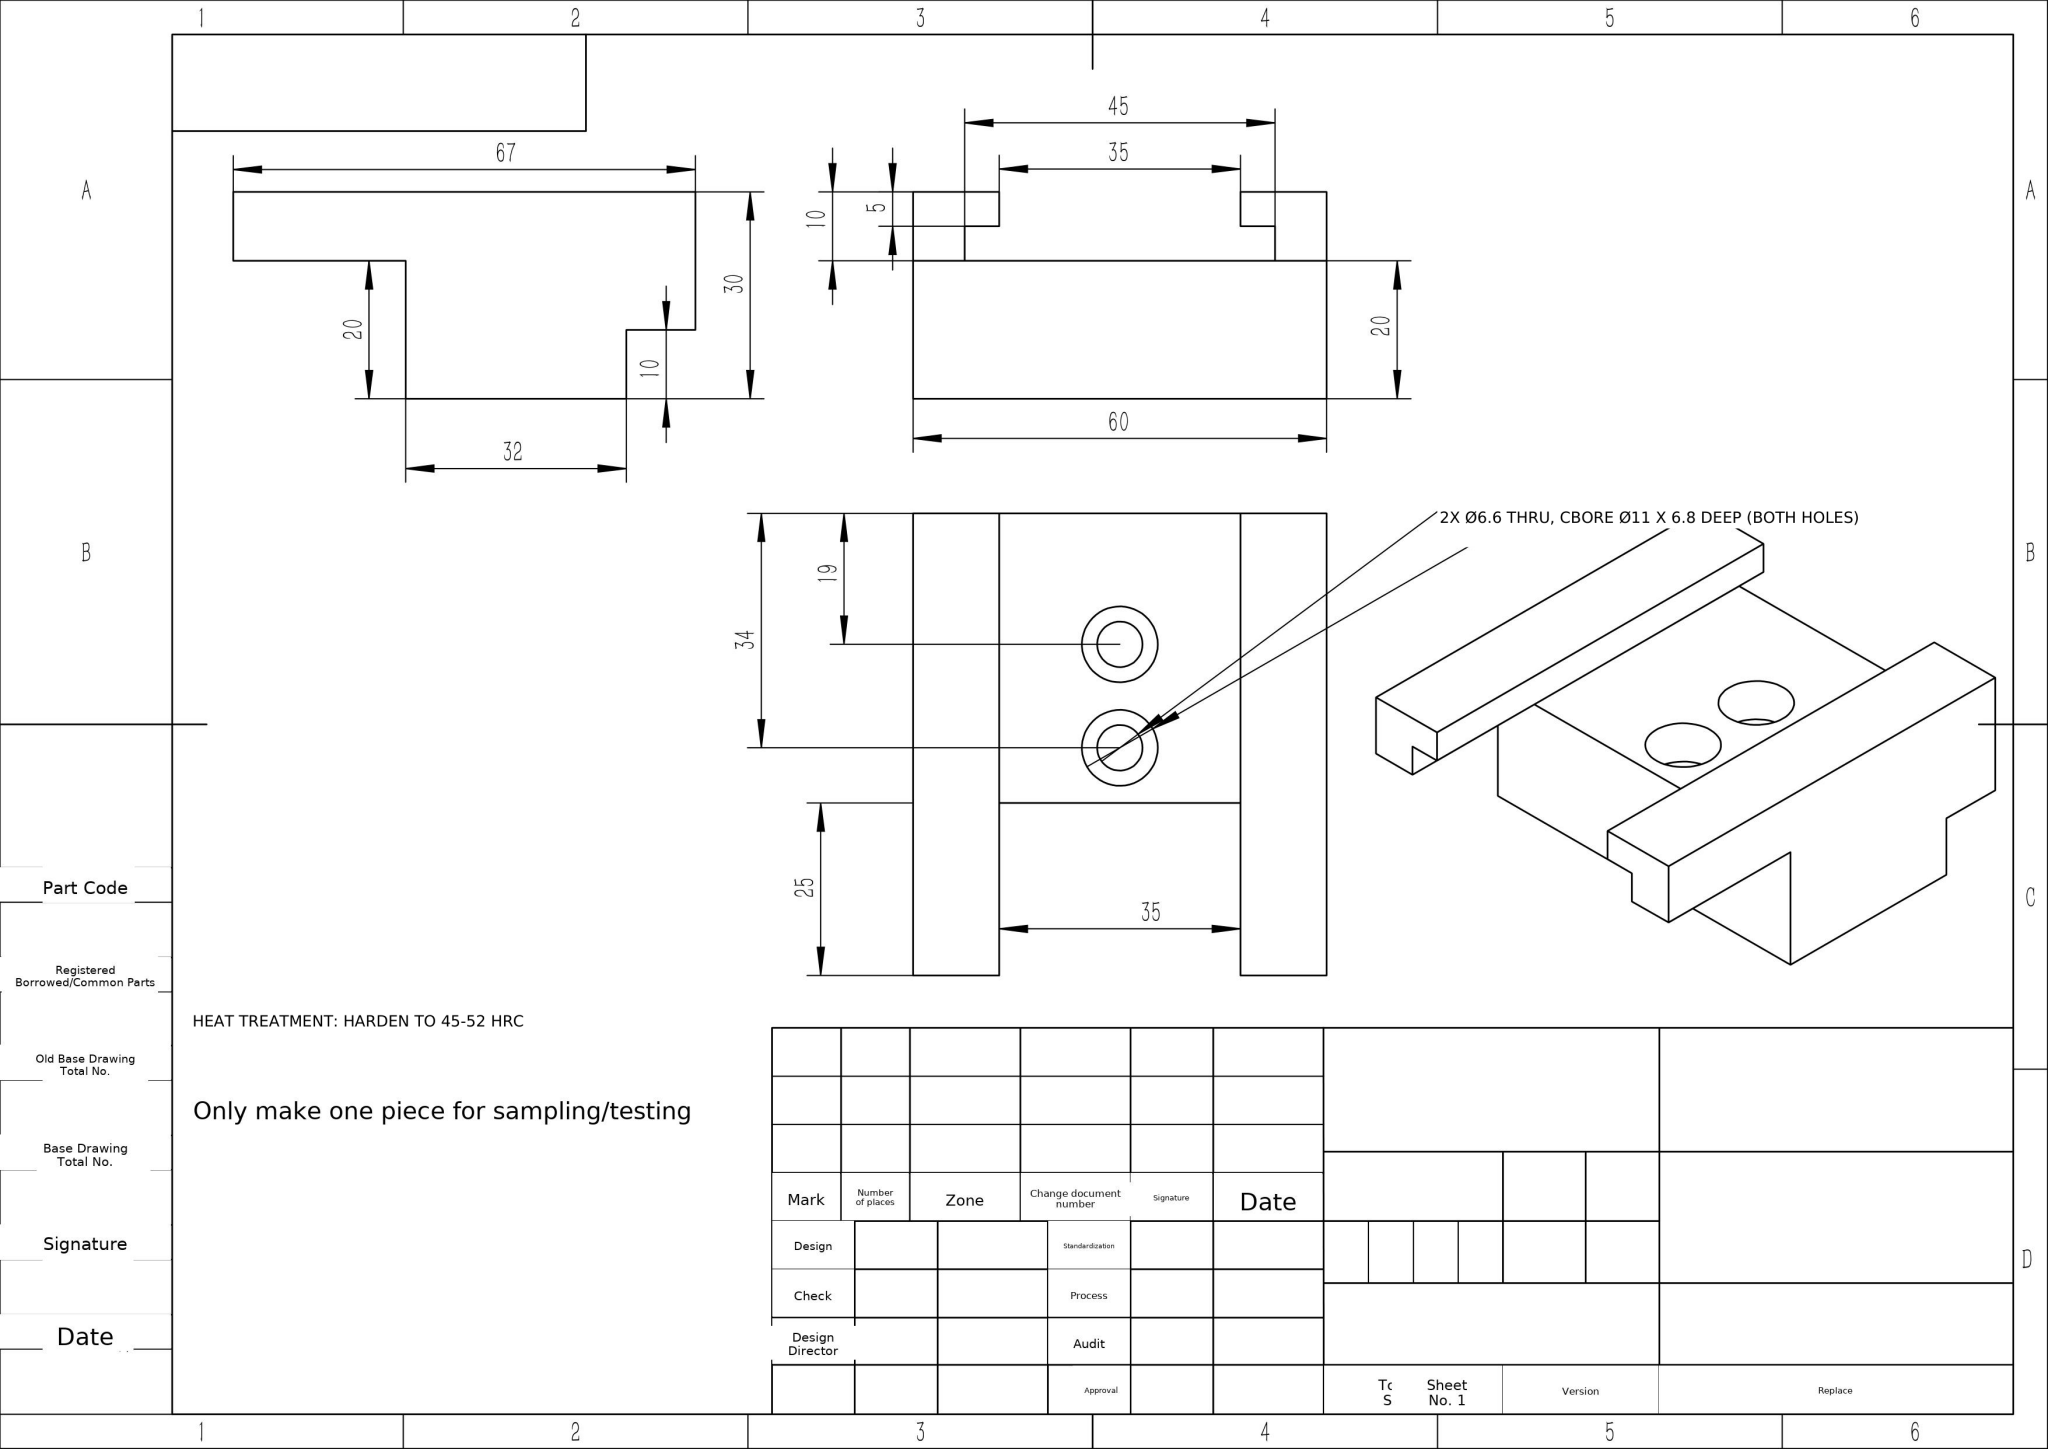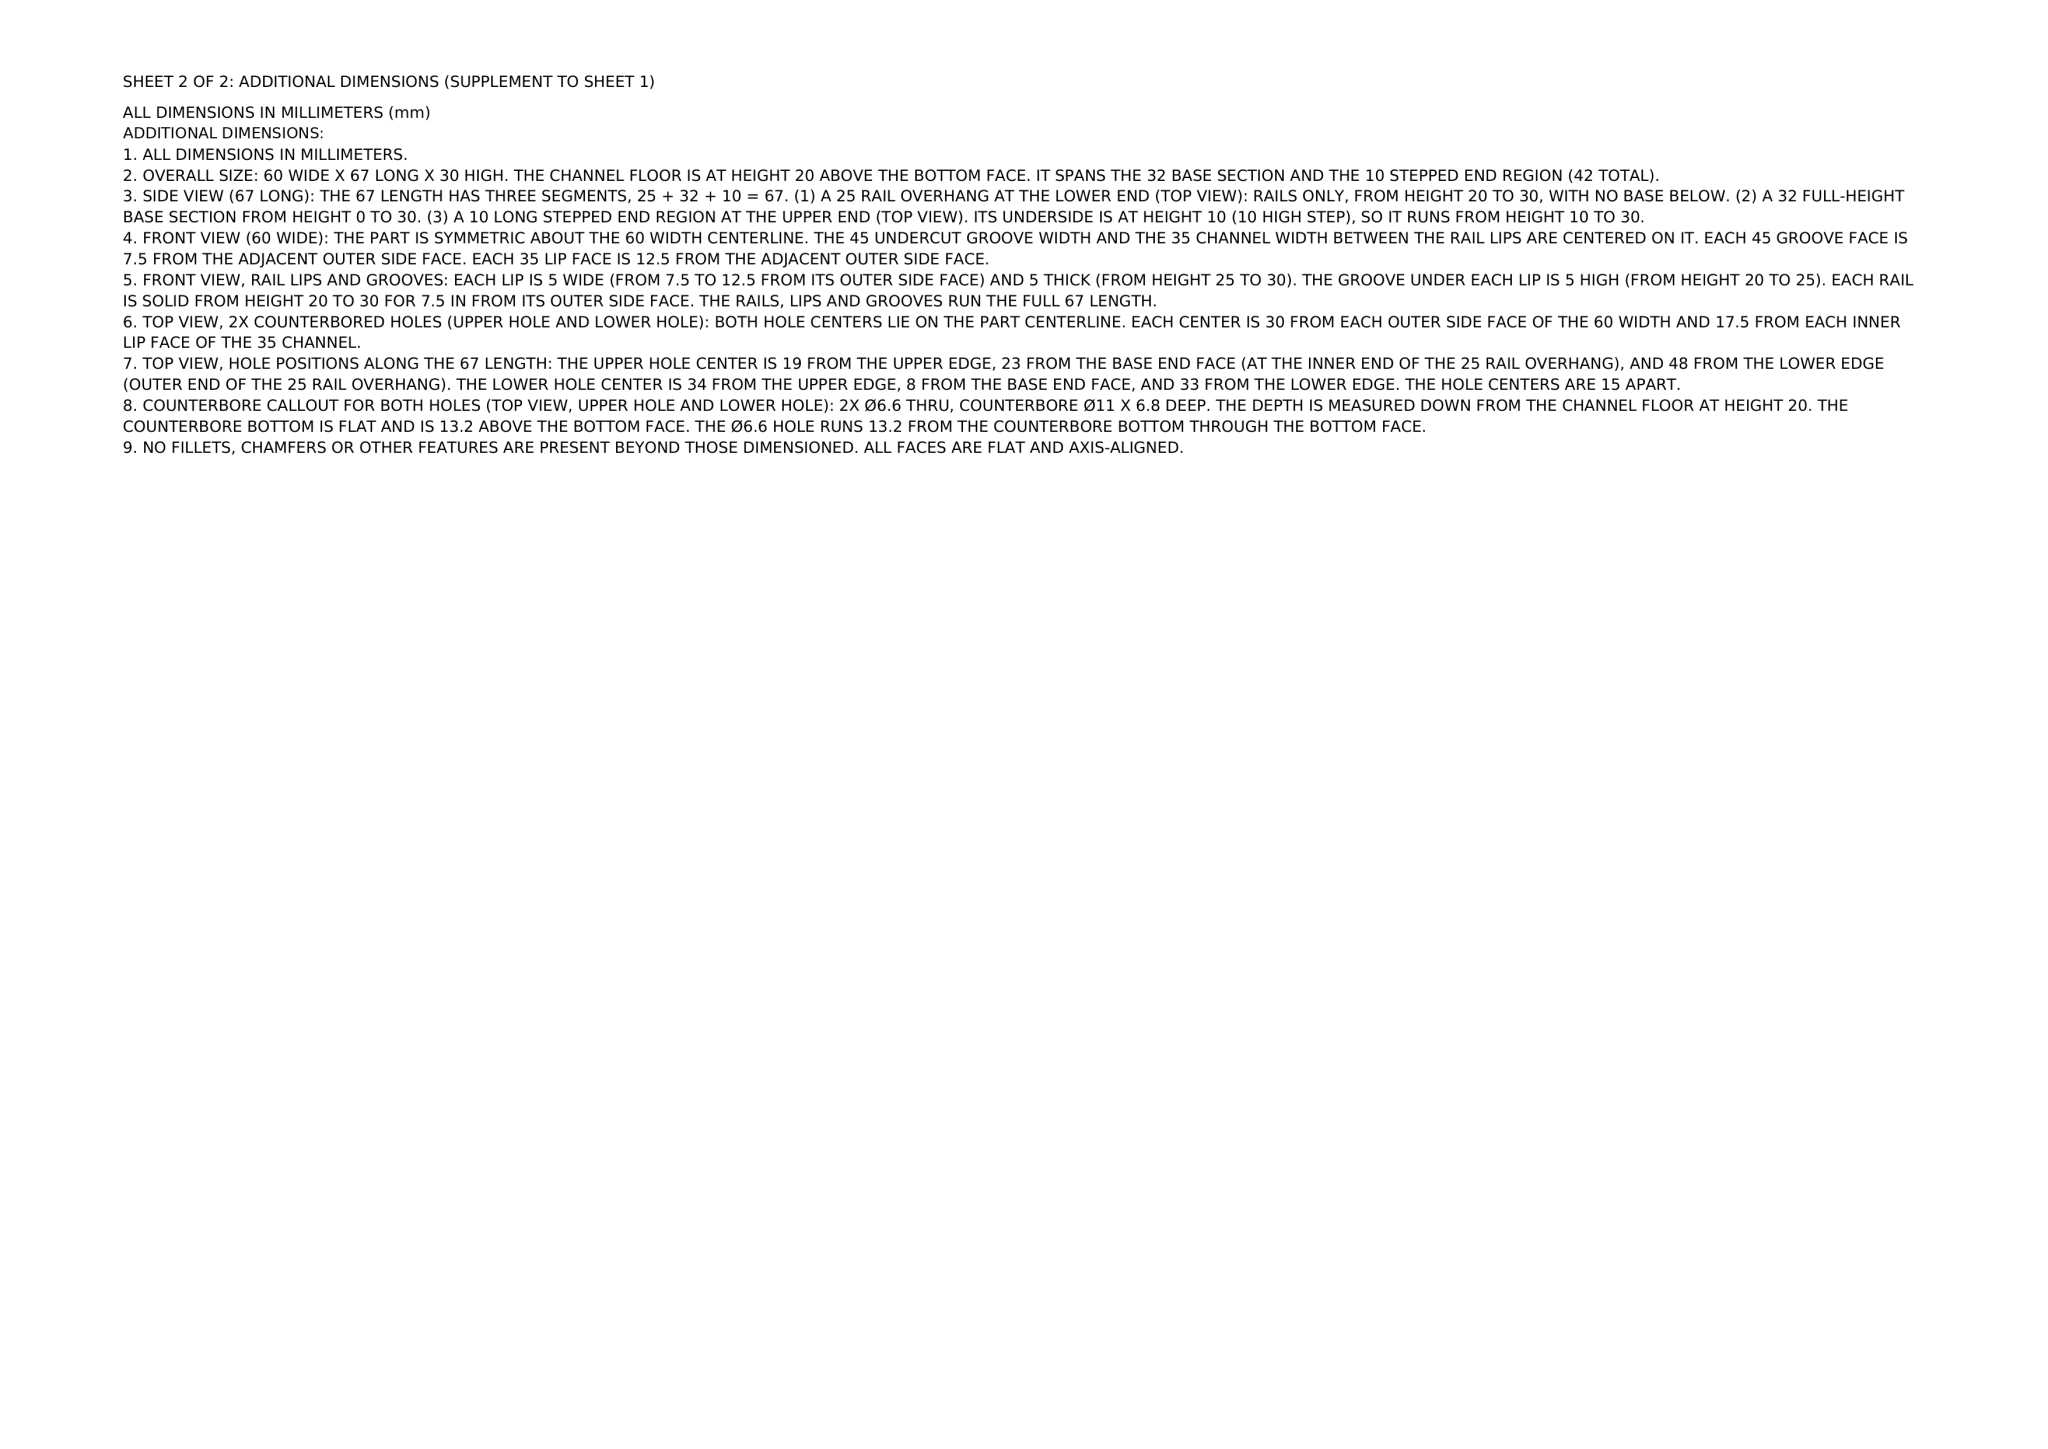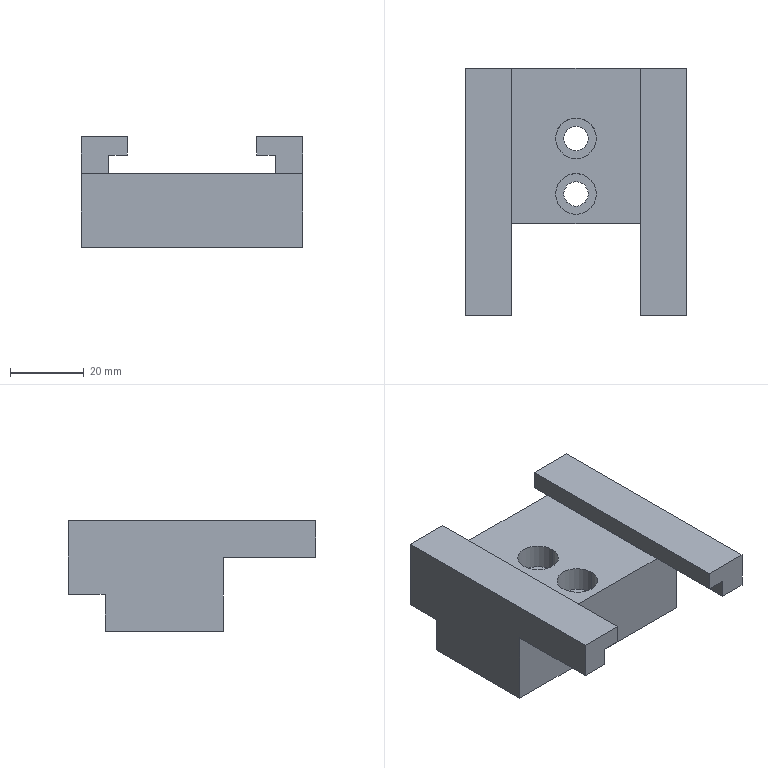Part | NX | mm | 1 solid | 30 faces | box 60 x 67 x 30 mm | volume 55604 mm3 | plane 22 | cylinder 8 | commonest cylinder face diameters 11 x4 6.6 x4